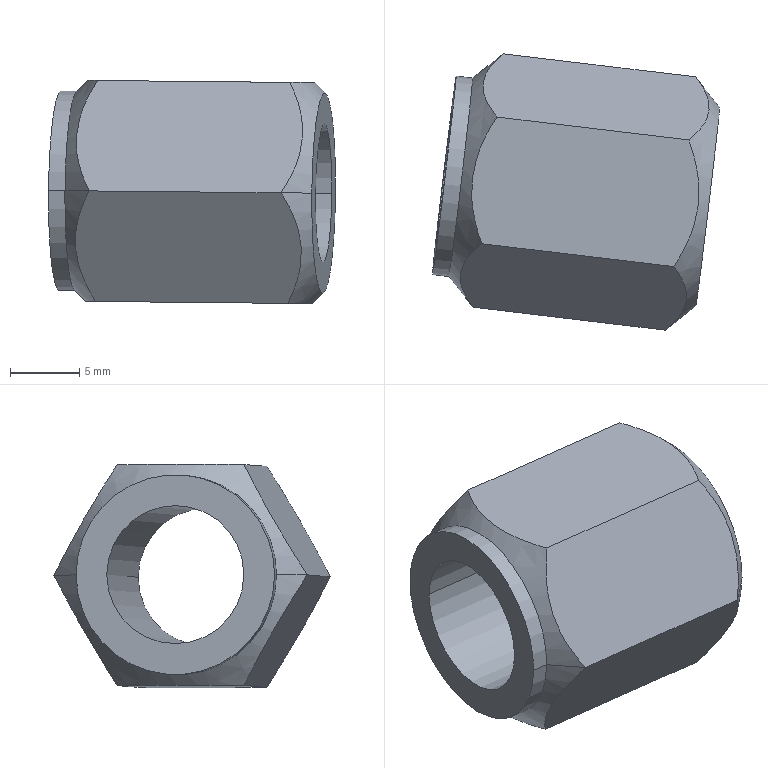Component | SolidWorks | Part13-1 | 1 solid | 16 faces | box 20.78 x 20 x 16.16 mm | volume 2605 mm3 | plane 8 | cone 4 | cylinder 4 | commonest cylinder face diameters 14.475 x2 10 x2 | material 45
build123d program:
from build123d import *

# Parameters (mm, degrees)
SKETCH2_R           = 5
BOSS_EXTRUDE1_DEPTH = 18
SKETCH4_R           = 7.238
SKETCH4_R_2         = 5
BOSS_EXTRUDE2_DEPTH = 1.2


with BuildPart() as part:
    # Sketch2 → Boss-Extrude1 (new body)
    with BuildSketch(Plane.XY):
        Polygon((6.238, 0), (1.619, 8), (-7.619, 8), (-12.238, 0), (-7.619, -8), (1.619, -8), align=None)
        with Locations((-3, 0)):
            Circle(SKETCH2_R, mode=Mode.SUBTRACT)
    extrude(amount=BOSS_EXTRUDE1_DEPTH)

    # Sketch3 → Cut-Revolve1 (revolve, cut)
    with BuildSketch(Plane(origin=(0, 0, 0), x_dir=(1, 0, 0), z_dir=(0, 1, 0)), mode=Mode.PRIVATE) as cut_revolve1_sk:
        Polygon((6.238, -16), (4.238, -18), (6.238, -18), align=None)
    revolve(cut_revolve1_sk.sketch.rotate(Axis((-3, 0, 18), (0, 0, 1)), 180), axis=Axis((-3, 0, 18), (0, 0, 1)), mode=Mode.SUBTRACT)

    # Sketch4 → Boss-Extrude2 (add)
    with BuildSketch(Plane.XY.offset(18)):
        with Locations((-3, 0)):
            Circle(SKETCH4_R)
        with Locations((-3, 0)):
            Circle(SKETCH4_R_2, mode=Mode.SUBTRACT)
    extrude(amount=BOSS_EXTRUDE2_DEPTH)

    # Sketch5 → Cut-Revolve2 (revolve, cut)
    with BuildSketch(Plane(origin=(0, 0, 0), x_dir=(1, 0, 0), z_dir=(0, 1, 0))):
        Polygon((4.238, 0), (6.238, 0), (6.238, -2), align=None)
    revolve(axis=Axis((-3, 0, 0), (0, 0, 1)), mode=Mode.SUBTRACT)


solid = part.part

# Placed as in the assembly
solid = solid.moved(Location((-11.695, 65.586, -1.735), (-85.302, -83.182, -175.339)))
STEP:
#1=COLOUR_RGB('',0.7922,0.8196,0.9333);
#2=FILL_AREA_STYLE_COLOUR('',#1);
#3=FILL_AREA_STYLE('',(#2));
#4=SURFACE_STYLE_FILL_AREA(#3);
#5=SURFACE_SIDE_STYLE('',(#4));
#6=SURFACE_STYLE_USAGE(.BOTH.,#5);
#7=PRESENTATION_STYLE_ASSIGNMENT((#6));
#8=CARTESIAN_POINT('',(-0.4802,2.416,-0.06797));
#9=VERTEX_POINT('',#8);
#10=CARTESIAN_POINT('',(-0.4127,2.982,-0.06863));
#11=VERTEX_POINT('',#10);
#12=CARTESIAN_POINT('',(-0.4465,2.699,-0.0683));
#13=DIRECTION('',(0.9929,-0.1183,-0.009724));
#14=DIRECTION('',(-0.1183,-0.993,0.001159));
#15=AXIS2_PLACEMENT_3D('',#12,#13,#14);
#16=CIRCLE('',#15,0.2849);
#17=EDGE_CURVE('',#9,#11,#16,.T.);
#18=ORIENTED_EDGE('',*,*,#17,.F.);
#19=CARTESIAN_POINT('',(-0.5677,2.348,-0.06712));
#20=VERTEX_POINT('',#19);
#21=CARTESIAN_POINT('',(-0.4802,2.416,-0.06797));
#22=DIRECTION('',(-0.7858,-0.6185,0.007696));
#23=VECTOR('',#22,39.37);
#24=LINE('',#21,#23);
#25=EDGE_CURVE('',#9,#20,#24,.T.);
#26=ORIENTED_EDGE('',*,*,#25,.T.);
#27=CARTESIAN_POINT('',(-0.5492,2.528,-0.3823));
#28=VERTEX_POINT('',#27);
#29=CARTESIAN_POINT('',(-0.5677,2.348,-0.06712));
#30=CARTESIAN_POINT('',(-0.5521,2.36,-0.09188));
#31=CARTESIAN_POINT('',(-0.5387,2.373,-0.1172));
#32=CARTESIAN_POINT('',(-0.5235,2.394,-0.1564));
#33=CARTESIAN_POINT('',(-0.5193,2.401,-0.1697));
#34=CARTESIAN_POINT('',(-0.513,2.416,-0.1969));
#35=CARTESIAN_POINT('',(-0.511,2.424,-0.2108));
#36=CARTESIAN_POINT('',(-0.5084,2.448,-0.2521));
#37=CARTESIAN_POINT('',(-0.5116,2.464,-0.2791));
#38=CARTESIAN_POINT('',(-0.5258,2.496,-0.3323));
#39=CARTESIAN_POINT('',(-0.5365,2.512,-0.3576));
#40=CARTESIAN_POINT('',(-0.5492,2.528,-0.3823));
#41=B_SPLINE_CURVE_WITH_KNOTS('',3,(#29,#30,#31,#32,#33,#34,#35,#36,#37,#38,#39,#40),.UNSPECIFIED.,.F.,.F.,(4,2,2,2,2,4),(0.00000025,0.002386,0.003579,0.004771,0.007157,0.009542),.UNSPECIFIED.);
#42=EDGE_CURVE('',#20,#28,#41,.T.);
#43=ORIENTED_EDGE('',*,*,#42,.T.);
#44=CARTESIAN_POINT('',(-0.5062,2.889,-0.3827));
#45=VERTEX_POINT('',#44);
#46=CARTESIAN_POINT('',(-0.5492,2.528,-0.3823));
#47=CARTESIAN_POINT('',(-0.5406,2.541,-0.3824));
#48=CARTESIAN_POINT('',(-0.5323,2.555,-0.3824));
#49=CARTESIAN_POINT('',(-0.5171,2.583,-0.3826));
#50=CARTESIAN_POINT('',(-0.51,2.597,-0.3827));
#51=CARTESIAN_POINT('',(-0.4979,2.626,-0.3828));
#52=CARTESIAN_POINT('',(-0.4926,2.641,-0.3828));
#53=CARTESIAN_POINT('',(-0.4843,2.671,-0.3829));
#54=CARTESIAN_POINT('',(-0.4812,2.687,-0.3829));
#55=CARTESIAN_POINT('',(-0.4756,2.735,-0.383));
#56=CARTESIAN_POINT('',(-0.4768,2.766,-0.383));
#57=CARTESIAN_POINT('',(-0.4843,2.813,-0.3829));
#58=CARTESIAN_POINT('',(-0.4878,2.829,-0.3829));
#59=CARTESIAN_POINT('',(-0.4961,2.859,-0.3828));
#60=CARTESIAN_POINT('',(-0.5009,2.874,-0.3827));
#61=CARTESIAN_POINT('',(-0.5062,2.889,-0.3827));
#62=B_SPLINE_CURVE_WITH_KNOTS('',3,(#46,#47,#48,#49,#50,#51,#52,#53,#54,#55,#56,#57,#58,#59,#60,#61),.UNSPECIFIED.,.F.,.F.,(4,2,2,2,2,2,2,4),(0.005616,0.006813,0.00801,0.009206,0.0104,0.0128,0.01399,0.01519),.UNSPECIFIED.);
#63=EDGE_CURVE('',#28,#45,#62,.T.);
#64=ORIENTED_EDGE('',*,*,#63,.T.);
#65=CARTESIAN_POINT('',(-0.4816,3.07,-0.06796));
#66=VERTEX_POINT('',#65);
#67=CARTESIAN_POINT('',(-0.5062,2.889,-0.3827));
#68=CARTESIAN_POINT('',(-0.4902,2.902,-0.3582));
#69=CARTESIAN_POINT('',(-0.4762,2.915,-0.3332));
#70=CARTESIAN_POINT('',(-0.4603,2.936,-0.2943));
#71=CARTESIAN_POINT('',(-0.4559,2.943,-0.2811));
#72=CARTESIAN_POINT('',(-0.449,2.958,-0.254));
#73=CARTESIAN_POINT('',(-0.4467,2.966,-0.2401));
#74=CARTESIAN_POINT('',(-0.4434,2.989,-0.1989));
#75=CARTESIAN_POINT('',(-0.446,3.005,-0.1719));
#76=CARTESIAN_POINT('',(-0.4592,3.038,-0.1184));
#77=CARTESIAN_POINT('',(-0.4694,3.054,-0.09283));
#78=CARTESIAN_POINT('',(-0.4816,3.07,-0.06796));
#79=B_SPLINE_CURVE_WITH_KNOTS('',3,(#67,#68,#69,#70,#71,#72,#73,#74,#75,#76,#77,#78),.UNSPECIFIED.,.F.,.F.,(4,2,2,2,2,4),(0.00000025,0.002386,0.003579,0.004771,0.007157,0.009542),.UNSPECIFIED.);
#80=EDGE_CURVE('',#45,#66,#79,.T.);
#81=ORIENTED_EDGE('',*,*,#80,.T.);
#82=CARTESIAN_POINT('',(-0.4127,2.982,-0.06863));
#83=DIRECTION('',(-0.6184,0.7858,0.006057));
#84=VECTOR('',#83,39.37);
#85=LINE('',#82,#84);
#86=EDGE_CURVE('',#11,#66,#85,.T.);
#87=ORIENTED_EDGE('',*,*,#86,.F.);
#88=EDGE_LOOP('',(#18,#26,#43,#64,#81,#87));
#89=FACE_OUTER_BOUND('',#88,.T.);
#90=CARTESIAN_POINT('',(-0.4465,2.699,-0.0683));
#91=DIRECTION('',(-0.9929,0.1183,0.009724));
#92=DIRECTION('',(0.1183,0.993,-0.001159));
#93=AXIS2_PLACEMENT_3D('',#90,#91,#92);
#94=CONICAL_SURFACE('',#93,0.2849,0.7854);
#95=ADVANCED_FACE('',(#89),#94,.T.);
#96=CARTESIAN_POINT('',(-1.163,3.072,-0.06128));
#97=VERTEX_POINT('',#96);
#98=CARTESIAN_POINT('',(-1.231,2.506,-0.06062));
#99=VERTEX_POINT('',#98);
#100=CARTESIAN_POINT('',(-1.197,2.789,-0.06095));
#101=DIRECTION('',(-0.9929,0.1183,0.009724));
#102=DIRECTION('',(0.1183,0.993,-0.001159));
#103=AXIS2_PLACEMENT_3D('',#100,#101,#102);
#104=CIRCLE('',#103,0.2849);
#105=EDGE_CURVE('',#97,#99,#104,.T.);
#106=ORIENTED_EDGE('',*,*,#105,.F.);
#107=CARTESIAN_POINT('',(-1.116,3.066,-0.06174));
#108=VERTEX_POINT('',#107);
#109=CARTESIAN_POINT('',(-1.163,3.072,-0.06128));
#110=DIRECTION('',(0.9929,-0.1183,-0.009724));
#111=VECTOR('',#110,39.37);
#112=LINE('',#109,#111);
#113=EDGE_CURVE('',#97,#108,#112,.T.);
#114=ORIENTED_EDGE('',*,*,#113,.T.);
#115=CARTESIAN_POINT('',(-1.184,2.5,-0.06108));
#116=VERTEX_POINT('',#115);
#117=CARTESIAN_POINT('',(-1.15,2.783,-0.06141));
#118=DIRECTION('',(-0.9929,0.1183,0.009724));
#119=DIRECTION('',(0.1183,0.993,-0.001159));
#120=AXIS2_PLACEMENT_3D('',#117,#118,#119);
#121=CIRCLE('',#120,0.2849);
#122=EDGE_CURVE('',#108,#116,#121,.T.);
#123=ORIENTED_EDGE('',*,*,#122,.T.);
#124=CARTESIAN_POINT('',(-1.231,2.506,-0.06062));
#125=DIRECTION('',(0.9929,-0.1183,-0.009724));
#126=VECTOR('',#125,39.37);
#127=LINE('',#124,#126);
#128=EDGE_CURVE('',#99,#116,#127,.T.);
#129=ORIENTED_EDGE('',*,*,#128,.F.);
#130=EDGE_LOOP('',(#106,#114,#123,#129));
#131=FACE_OUTER_BOUND('',#130,.T.);
#132=CARTESIAN_POINT('',(-1.197,2.789,-0.06095));
#133=DIRECTION('',(0.9929,-0.1183,-0.009724));
#134=DIRECTION('',(-0.1183,-0.993,0.001159));
#135=AXIS2_PLACEMENT_3D('',#132,#133,#134);
#136=CYLINDRICAL_SURFACE('',#135,0.2849);
#137=ADVANCED_FACE('',(#131),#136,.T.);
#138=ORIENTED_EDGE('',*,*,#122,.F.);
#139=CARTESIAN_POINT('',(-1.029,3.135,-0.0626));
#140=VERTEX_POINT('',#139);
#141=CARTESIAN_POINT('',(-1.029,3.135,-0.0626));
#142=DIRECTION('',(0.7858,0.6185,-0.007696));
#143=VECTOR('',#142,39.37);
#144=LINE('',#141,#143);
#145=EDGE_CURVE('',#108,#140,#144,.T.);
#146=ORIENTED_EDGE('',*,*,#145,.T.);
#147=CARTESIAN_POINT('',(-1.053,2.954,-0.3773));
#148=VERTEX_POINT('',#147);
#149=CARTESIAN_POINT('',(-1.029,3.135,-0.0626));
#150=CARTESIAN_POINT('',(-1.045,3.123,-0.08705));
#151=CARTESIAN_POINT('',(-1.059,3.11,-0.1121));
#152=CARTESIAN_POINT('',(-1.075,3.089,-0.151));
#153=CARTESIAN_POINT('',(-1.079,3.082,-0.1642));
#154=CARTESIAN_POINT('',(-1.086,3.067,-0.1913));
#155=CARTESIAN_POINT('',(-1.088,3.059,-0.2052));
#156=CARTESIAN_POINT('',(-1.092,3.035,-0.2464));
#157=CARTESIAN_POINT('',(-1.089,3.019,-0.2734));
#158=CARTESIAN_POINT('',(-1.076,2.986,-0.3269));
#159=CARTESIAN_POINT('',(-1.066,2.97,-0.3525));
#160=CARTESIAN_POINT('',(-1.053,2.954,-0.3773));
#161=B_SPLINE_CURVE_WITH_KNOTS('',3,(#149,#150,#151,#152,#153,#154,#155,#156,#157,#158,#159,#160),.UNSPECIFIED.,.F.,.F.,(4,2,2,2,2,4),(0.00000025,0.002386,0.003579,0.004771,0.007157,0.009542),.UNSPECIFIED.);
#162=EDGE_CURVE('',#140,#148,#161,.T.);
#163=ORIENTED_EDGE('',*,*,#162,.T.);
#164=CARTESIAN_POINT('',(-1.097,2.593,-0.3769));
#165=VERTEX_POINT('',#164);
#166=CARTESIAN_POINT('',(-1.053,2.954,-0.3773));
#167=CARTESIAN_POINT('',(-1.062,2.941,-0.3772));
#168=CARTESIAN_POINT('',(-1.07,2.928,-0.3772));
#169=CARTESIAN_POINT('',(-1.086,2.9,-0.377));
#170=CARTESIAN_POINT('',(-1.093,2.886,-0.3769));
#171=CARTESIAN_POINT('',(-1.111,2.842,-0.3768));
#172=CARTESIAN_POINT('',(-1.12,2.812,-0.3767));
#173=CARTESIAN_POINT('',(-1.125,2.764,-0.3766));
#174=CARTESIAN_POINT('',(-1.126,2.748,-0.3766));
#175=CARTESIAN_POINT('',(-1.125,2.716,-0.3766));
#176=CARTESIAN_POINT('',(-1.123,2.701,-0.3766));
#177=CARTESIAN_POINT('',(-1.118,2.67,-0.3767));
#178=CARTESIAN_POINT('',(-1.115,2.654,-0.3767));
#179=CARTESIAN_POINT('',(-1.107,2.623,-0.3768));
#180=CARTESIAN_POINT('',(-1.102,2.608,-0.3769));
#181=CARTESIAN_POINT('',(-1.097,2.593,-0.3769));
#182=B_SPLINE_CURVE_WITH_KNOTS('',3,(#166,#167,#168,#169,#170,#171,#172,#173,#174,#175,#176,#177,#178,#179,#180,#181),.UNSPECIFIED.,.F.,.F.,(4,2,2,2,2,2,2,4),(0.004981,0.006177,0.007373,0.009765,0.01096,0.01216,0.01335,0.01455),.UNSPECIFIED.);
#183=EDGE_CURVE('',#148,#165,#182,.T.);
#184=ORIENTED_EDGE('',*,*,#183,.T.);
#185=CARTESIAN_POINT('',(-1.115,2.413,-0.06176));
#186=VERTEX_POINT('',#185);
#187=CARTESIAN_POINT('',(-1.097,2.593,-0.3769));
#188=CARTESIAN_POINT('',(-1.112,2.581,-0.3521));
#189=CARTESIAN_POINT('',(-1.126,2.568,-0.3269));
#190=CARTESIAN_POINT('',(-1.141,2.547,-0.2876));
#191=CARTESIAN_POINT('',(-1.145,2.54,-0.2743));
#192=CARTESIAN_POINT('',(-1.151,2.525,-0.2472));
#193=CARTESIAN_POINT('',(-1.153,2.517,-0.2332));
#194=CARTESIAN_POINT('',(-1.156,2.493,-0.1919));
#195=CARTESIAN_POINT('',(-1.153,2.477,-0.1649));
#196=CARTESIAN_POINT('',(-1.138,2.445,-0.1118));
#197=CARTESIAN_POINT('',(-1.128,2.429,-0.08639));
#198=CARTESIAN_POINT('',(-1.115,2.413,-0.06176));
#199=B_SPLINE_CURVE_WITH_KNOTS('',3,(#187,#188,#189,#190,#191,#192,#193,#194,#195,#196,#197,#198),.UNSPECIFIED.,.F.,.F.,(4,2,2,2,2,4),(0.00000025,0.002386,0.003579,0.004771,0.007157,0.009542),.UNSPECIFIED.);
#200=EDGE_CURVE('',#165,#186,#199,.T.);
#201=ORIENTED_EDGE('',*,*,#200,.T.);
#202=CARTESIAN_POINT('',(-1.115,2.413,-0.06176));
#203=DIRECTION('',(0.6184,-0.7858,-0.006057));
#204=VECTOR('',#203,39.37);
#205=LINE('',#202,#204);
#206=EDGE_CURVE('',#116,#186,#205,.T.);
#207=ORIENTED_EDGE('',*,*,#206,.F.);
#208=EDGE_LOOP('',(#138,#146,#163,#184,#201,#207));
#209=FACE_OUTER_BOUND('',#208,.T.);
#210=CARTESIAN_POINT('',(-1.072,2.774,-0.06218));
#211=DIRECTION('',(0.9929,-0.1183,-0.009724));
#212=DIRECTION('',(-0.1183,-0.993,0.001159));
#213=AXIS2_PLACEMENT_3D('',#210,#211,#212);
#214=CONICAL_SURFACE('',#213,0.3637,0.7854);
#215=ADVANCED_FACE('',(#209),#214,.T.);
#216=CARTESIAN_POINT('',(-1.22,2.593,-0.06072));
#217=VERTEX_POINT('',#216);
#218=CARTESIAN_POINT('',(-1.174,2.984,-0.06118));
#219=VERTEX_POINT('',#218);
#220=CARTESIAN_POINT('',(-1.197,2.789,-0.06095));
#221=DIRECTION('',(-0.9929,0.1183,0.009724));
#222=DIRECTION('',(0.1183,0.993,-0.001159));
#223=AXIS2_PLACEMENT_3D('',#220,#221,#222);
#224=CIRCLE('',#223,0.1969);
#225=EDGE_CURVE('',#217,#219,#224,.T.);
#226=ORIENTED_EDGE('',*,*,#225,.T.);
#227=CARTESIAN_POINT('',(-0.4232,2.895,-0.06853));
#228=VERTEX_POINT('',#227);
#229=CARTESIAN_POINT('',(-1.127,2.979,-0.06164));
#230=DIRECTION('',(0.9929,-0.1183,-0.009724));
#231=VECTOR('',#230,39.37);
#232=LINE('',#229,#231);
#233=EDGE_CURVE('',#219,#228,#232,.T.);
#234=ORIENTED_EDGE('',*,*,#233,.T.);
#235=CARTESIAN_POINT('',(-0.4698,2.504,-0.06807));
#236=VERTEX_POINT('',#235);
#237=CARTESIAN_POINT('',(-0.4465,2.699,-0.0683));
#238=DIRECTION('',(-0.9929,0.1183,0.009724));
#239=DIRECTION('',(0.1183,0.993,-0.001159));
#240=AXIS2_PLACEMENT_3D('',#237,#238,#239);
#241=CIRCLE('',#240,0.1969);
#242=EDGE_CURVE('',#236,#228,#241,.T.);
#243=ORIENTED_EDGE('',*,*,#242,.F.);
#244=CARTESIAN_POINT('',(-1.173,2.588,-0.06118));
#245=DIRECTION('',(0.9929,-0.1183,-0.009724));
#246=VECTOR('',#245,39.37);
#247=LINE('',#244,#246);
#248=EDGE_CURVE('',#217,#236,#247,.T.);
#249=ORIENTED_EDGE('',*,*,#248,.F.);
#250=EDGE_LOOP('',(#226,#234,#243,#249));
#251=FACE_OUTER_BOUND('',#250,.T.);
#252=CARTESIAN_POINT('',(-1.15,2.783,-0.06141));
#253=DIRECTION('',(0.9929,-0.1183,-0.009724));
#254=DIRECTION('',(-0.1183,-0.993,0.001159));
#255=AXIS2_PLACEMENT_3D('',#252,#253,#254);
#256=CYLINDRICAL_SURFACE('',#255,0.1969);
#257=ADVANCED_FACE('',(#251),#256,.F.);
#258=CARTESIAN_POINT('',(-0.5,2.889,0.2472));
#259=VERTEX_POINT('',#258);
#260=CARTESIAN_POINT('',(-0.4816,3.07,-0.06796));
#261=CARTESIAN_POINT('',(-0.4689,3.054,-0.04347));
#262=CARTESIAN_POINT('',(-0.4584,3.038,-0.01841));
#263=CARTESIAN_POINT('',(-0.4479,3.014,0.02058));
#264=CARTESIAN_POINT('',(-0.4452,3.006,0.03382));
#265=CARTESIAN_POINT('',(-0.4421,2.99,0.06087));
#266=CARTESIAN_POINT('',(-0.4416,2.982,0.07481));
#267=CARTESIAN_POINT('',(-0.444,2.958,0.1161));
#268=CARTESIAN_POINT('',(-0.4503,2.943,0.1432));
#269=CARTESIAN_POINT('',(-0.4707,2.915,0.1967));
#270=CARTESIAN_POINT('',(-0.4844,2.902,0.2223));
#271=CARTESIAN_POINT('',(-0.5,2.889,0.2472));
#272=B_SPLINE_CURVE_WITH_KNOTS('',3,(#260,#261,#262,#263,#264,#265,#266,#267,#268,#269,#270,#271),.UNSPECIFIED.,.F.,.F.,(4,2,2,2,2,4),(0.00000025,0.002386,0.003579,0.004771,0.007157,0.009542),.UNSPECIFIED.);
#273=EDGE_CURVE('',#66,#259,#272,.T.);
#274=ORIENTED_EDGE('',*,*,#273,.F.);
#275=CARTESIAN_POINT('',(-1.107,3.144,-0.06183));
#276=DIRECTION('',(0.9929,-0.1183,-0.009724));
#277=VECTOR('',#276,39.37);
#278=LINE('',#275,#277);
#279=EDGE_CURVE('',#140,#66,#278,.T.);
#280=ORIENTED_EDGE('',*,*,#279,.F.);
#281=CARTESIAN_POINT('',(-1.047,2.954,0.2526));
#282=VERTEX_POINT('',#281);
#283=CARTESIAN_POINT('',(-1.047,2.954,0.2526));
#284=CARTESIAN_POINT('',(-1.06,2.97,0.2281));
#285=CARTESIAN_POINT('',(-1.071,2.986,0.203));
#286=CARTESIAN_POINT('',(-1.081,3.01,0.164));
#287=CARTESIAN_POINT('',(-1.084,3.018,0.1508));
#288=CARTESIAN_POINT('',(-1.087,3.034,0.1237));
#289=CARTESIAN_POINT('',(-1.087,3.042,0.1098));
#290=CARTESIAN_POINT('',(-1.085,3.066,0.06852));
#291=CARTESIAN_POINT('',(-1.079,3.081,0.04143));
#292=CARTESIAN_POINT('',(-1.058,3.109,-0.01207));
#293=CARTESIAN_POINT('',(-1.045,3.123,-0.03769));
#294=CARTESIAN_POINT('',(-1.029,3.135,-0.0626));
#295=B_SPLINE_CURVE_WITH_KNOTS('',3,(#283,#284,#285,#286,#287,#288,#289,#290,#291,#292,#293,#294),.UNSPECIFIED.,.F.,.F.,(4,2,2,2,2,4),(0.00000025,0.002386,0.003579,0.004771,0.007157,0.009542),.UNSPECIFIED.);
#296=EDGE_CURVE('',#282,#140,#295,.T.);
#297=ORIENTED_EDGE('',*,*,#296,.F.);
#298=CARTESIAN_POINT('',(-1.126,2.964,0.2533));
#299=DIRECTION('',(0.9929,-0.1183,-0.009724));
#300=VECTOR('',#299,39.37);
#301=LINE('',#298,#300);
#302=EDGE_CURVE('',#282,#259,#301,.T.);
#303=ORIENTED_EDGE('',*,*,#302,.T.);
#304=EDGE_LOOP('',(#274,#280,#297,#303));
#305=FACE_OUTER_BOUND('',#304,.T.);
#306=CARTESIAN_POINT('',(-1.126,2.964,0.2533));
#307=DIRECTION('',(-0.1074,-0.8599,-0.499));
#308=DIRECTION('',(-0.05068,-0.4965,0.8666));
#309=AXIS2_PLACEMENT_3D('',#306,#307,#308);
#310=PLANE('',#309);
#311=ADVANCED_FACE('',(#305),#310,.F.);
#312=ORIENTED_EDGE('',*,*,#80,.F.);
#313=CARTESIAN_POINT('',(-1.132,2.964,-0.3766));
#314=DIRECTION('',(0.9929,-0.1183,-0.009724));
#315=VECTOR('',#314,39.37);
#316=LINE('',#313,#315);
#317=EDGE_CURVE('',#148,#45,#316,.T.);
#318=ORIENTED_EDGE('',*,*,#317,.F.);
#319=ORIENTED_EDGE('',*,*,#162,.F.);
#320=ORIENTED_EDGE('',*,*,#279,.T.);
#321=EDGE_LOOP('',(#312,#318,#319,#320));
#322=FACE_OUTER_BOUND('',#321,.T.);
#323=CARTESIAN_POINT('',(-1.107,3.144,-0.06183));
#324=DIRECTION('',(-0.09757,-0.8599,0.501));
#325=DIRECTION('',(0.06764,0.4965,0.8654));
#326=AXIS2_PLACEMENT_3D('',#323,#324,#325);
#327=PLANE('',#326);
#328=ADVANCED_FACE('',(#322),#327,.F.);
#329=ORIENTED_EDGE('',*,*,#63,.F.);
#330=CARTESIAN_POINT('',(-1.175,2.603,-0.3761));
#331=DIRECTION('',(0.9929,-0.1183,-0.009724));
#332=VECTOR('',#331,39.37);
#333=LINE('',#330,#332);
#334=EDGE_CURVE('',#165,#28,#333,.T.);
#335=ORIENTED_EDGE('',*,*,#334,.F.);
#336=ORIENTED_EDGE('',*,*,#183,.F.);
#337=ORIENTED_EDGE('',*,*,#317,.T.);
#338=EDGE_LOOP('',(#329,#335,#336,#337));
#339=FACE_OUTER_BOUND('',#338,.T.);
#340=CARTESIAN_POINT('',(-1.132,2.964,-0.3766));
#341=DIRECTION('',(0.009793,0.,1.));
#342=DIRECTION('',(0.9929,-0.1183,-0.009724));
#343=AXIS2_PLACEMENT_3D('',#340,#341,#342);
#344=PLANE('',#343);
#345=ADVANCED_FACE('',(#339),#344,.F.);
#346=ORIENTED_EDGE('',*,*,#42,.F.);
#347=CARTESIAN_POINT('',(-1.193,2.422,-0.06099));
#348=DIRECTION('',(0.9929,-0.1183,-0.009724));
#349=VECTOR('',#348,39.37);
#350=LINE('',#347,#349);
#351=EDGE_CURVE('',#186,#20,#350,.T.);
#352=ORIENTED_EDGE('',*,*,#351,.F.);
#353=ORIENTED_EDGE('',*,*,#200,.F.);
#354=ORIENTED_EDGE('',*,*,#334,.T.);
#355=EDGE_LOOP('',(#346,#352,#353,#354));
#356=FACE_OUTER_BOUND('',#355,.T.);
#357=CARTESIAN_POINT('',(-1.175,2.603,-0.3761));
#358=DIRECTION('',(0.1074,0.8599,0.499));
#359=DIRECTION('',(0.05068,0.4965,-0.8666));
#360=AXIS2_PLACEMENT_3D('',#357,#358,#359);
#361=PLANE('',#360);
#362=ADVANCED_FACE('',(#356),#361,.F.);
#363=CARTESIAN_POINT('',(-0.5431,2.528,0.2476));
#364=VERTEX_POINT('',#363);
#365=CARTESIAN_POINT('',(-0.5431,2.528,0.2476));
#366=CARTESIAN_POINT('',(-0.5309,2.512,0.2229));
#367=CARTESIAN_POINT('',(-0.5209,2.497,0.1976));
#368=CARTESIAN_POINT('',(-0.5111,2.473,0.1584));
#369=CARTESIAN_POINT('',(-0.5087,2.465,0.1451));
#370=CARTESIAN_POINT('',(-0.5061,2.448,0.118));
#371=CARTESIAN_POINT('',(-0.5059,2.44,0.1041));
#372=CARTESIAN_POINT('',(-0.509,2.417,0.06288));
#373=CARTESIAN_POINT('',(-0.5159,2.402,0.03592));
#374=CARTESIAN_POINT('',(-0.5374,2.373,-0.01717));
#375=CARTESIAN_POINT('',(-0.5516,2.36,-0.04252));
#376=CARTESIAN_POINT('',(-0.5677,2.348,-0.06712));
#377=B_SPLINE_CURVE_WITH_KNOTS('',3,(#365,#366,#367,#368,#369,#370,#371,#372,#373,#374,#375,#376),.UNSPECIFIED.,.F.,.F.,(4,2,2,2,2,4),(0.00000025,0.002386,0.003579,0.004771,0.007157,0.009542),.UNSPECIFIED.);
#378=EDGE_CURVE('',#364,#20,#377,.T.);
#379=ORIENTED_EDGE('',*,*,#378,.F.);
#380=CARTESIAN_POINT('',(-1.09,2.593,0.253));
#381=VERTEX_POINT('',#380);
#382=CARTESIAN_POINT('',(-1.169,2.603,0.2537));
#383=DIRECTION('',(0.9929,-0.1183,-0.009724));
#384=VECTOR('',#383,39.37);
#385=LINE('',#382,#384);
#386=EDGE_CURVE('',#381,#364,#385,.T.);
#387=ORIENTED_EDGE('',*,*,#386,.F.);
#388=CARTESIAN_POINT('',(-1.115,2.413,-0.06176));
#389=CARTESIAN_POINT('',(-1.127,2.429,-0.03703));
#390=CARTESIAN_POINT('',(-1.137,2.444,-0.01176));
#391=CARTESIAN_POINT('',(-1.147,2.468,0.02743));
#392=CARTESIAN_POINT('',(-1.149,2.476,0.04071));
#393=CARTESIAN_POINT('',(-1.152,2.492,0.06782));
#394=CARTESIAN_POINT('',(-1.152,2.501,0.08177));
#395=CARTESIAN_POINT('',(-1.149,2.524,0.123));
#396=CARTESIAN_POINT('',(-1.142,2.539,0.1499));
#397=CARTESIAN_POINT('',(-1.121,2.568,0.203));
#398=CARTESIAN_POINT('',(-1.106,2.581,0.2284));
#399=CARTESIAN_POINT('',(-1.09,2.593,0.253));
#400=B_SPLINE_CURVE_WITH_KNOTS('',3,(#388,#389,#390,#391,#392,#393,#394,#395,#396,#397,#398,#399),.UNSPECIFIED.,.F.,.F.,(4,2,2,2,2,4),(0.00000025,0.002386,0.003579,0.004771,0.007157,0.009542),.UNSPECIFIED.);
#401=EDGE_CURVE('',#186,#381,#400,.T.);
#402=ORIENTED_EDGE('',*,*,#401,.F.);
#403=ORIENTED_EDGE('',*,*,#351,.T.);
#404=EDGE_LOOP('',(#379,#387,#402,#403));
#405=FACE_OUTER_BOUND('',#404,.T.);
#406=CARTESIAN_POINT('',(-1.193,2.422,-0.06099));
#407=DIRECTION('',(0.09757,0.8599,-0.501));
#408=DIRECTION('',(-0.06764,-0.4965,-0.8654));
#409=AXIS2_PLACEMENT_3D('',#406,#407,#408);
#410=PLANE('',#409);
#411=ADVANCED_FACE('',(#405),#410,.F.);
#412=CARTESIAN_POINT('',(-0.5,2.889,0.2472));
#413=CARTESIAN_POINT('',(-0.4947,2.874,0.2471));
#414=CARTESIAN_POINT('',(-0.4899,2.859,0.2471));
#415=CARTESIAN_POINT('',(-0.4816,2.829,0.247));
#416=CARTESIAN_POINT('',(-0.4781,2.813,0.247));
#417=CARTESIAN_POINT('',(-0.4706,2.766,0.2469));
#418=CARTESIAN_POINT('',(-0.4694,2.735,0.2469));
#419=CARTESIAN_POINT('',(-0.4751,2.687,0.247));
#420=CARTESIAN_POINT('',(-0.4782,2.671,0.247));
#421=CARTESIAN_POINT('',(-0.4865,2.641,0.2471));
#422=CARTESIAN_POINT('',(-0.4917,2.626,0.2471));
#423=CARTESIAN_POINT('',(-0.5039,2.597,0.2472));
#424=CARTESIAN_POINT('',(-0.5109,2.583,0.2473));
#425=CARTESIAN_POINT('',(-0.5262,2.555,0.2475));
#426=CARTESIAN_POINT('',(-0.5344,2.541,0.2475));
#427=CARTESIAN_POINT('',(-0.5431,2.528,0.2476));
#428=B_SPLINE_CURVE_WITH_KNOTS('',3,(#412,#413,#414,#415,#416,#417,#418,#419,#420,#421,#422,#423,#424,#425,#426,#427),.UNSPECIFIED.,.F.,.F.,(4,2,2,2,2,2,2,4),(0.004981,0.006177,0.007373,0.009765,0.01096,0.01216,0.01335,0.01455),.UNSPECIFIED.);
#429=EDGE_CURVE('',#259,#364,#428,.T.);
#430=ORIENTED_EDGE('',*,*,#429,.F.);
#431=ORIENTED_EDGE('',*,*,#302,.F.);
#432=CARTESIAN_POINT('',(-1.09,2.593,0.253));
#433=CARTESIAN_POINT('',(-1.096,2.608,0.253));
#434=CARTESIAN_POINT('',(-1.101,2.623,0.2531));
#435=CARTESIAN_POINT('',(-1.109,2.654,0.2532));
#436=CARTESIAN_POINT('',(-1.112,2.67,0.2532));
#437=CARTESIAN_POINT('',(-1.117,2.701,0.2532));
#438=CARTESIAN_POINT('',(-1.119,2.716,0.2533));
#439=CARTESIAN_POINT('',(-1.12,2.748,0.2533));
#440=CARTESIAN_POINT('',(-1.119,2.764,0.2533));
#441=CARTESIAN_POINT('',(-1.113,2.812,0.2532));
#442=CARTESIAN_POINT('',(-1.105,2.842,0.2531));
#443=CARTESIAN_POINT('',(-1.086,2.886,0.2529));
#444=CARTESIAN_POINT('',(-1.079,2.9,0.2529));
#445=CARTESIAN_POINT('',(-1.064,2.928,0.2527));
#446=CARTESIAN_POINT('',(-1.056,2.941,0.2526));
#447=CARTESIAN_POINT('',(-1.047,2.954,0.2526));
#448=B_SPLINE_CURVE_WITH_KNOTS('',3,(#432,#433,#434,#435,#436,#437,#438,#439,#440,#441,#442,#443,#444,#445,#446,#447),.UNSPECIFIED.,.F.,.F.,(4,2,2,2,2,2,2,4),(0.005616,0.006813,0.00801,0.009206,0.0104,0.0128,0.01399,0.01519),.UNSPECIFIED.);
#449=EDGE_CURVE('',#381,#282,#448,.T.);
#450=ORIENTED_EDGE('',*,*,#449,.F.);
#451=ORIENTED_EDGE('',*,*,#386,.T.);
#452=EDGE_LOOP('',(#430,#431,#450,#451));
#453=FACE_OUTER_BOUND('',#452,.T.);
#454=CARTESIAN_POINT('',(-1.169,2.603,0.2537));
#455=DIRECTION('',(-0.009793,-0.,-1.));
#456=DIRECTION('',(-0.9929,0.1183,0.009724));
#457=AXIS2_PLACEMENT_3D('',#454,#455,#456);
#458=PLANE('',#457);
#459=ADVANCED_FACE('',(#453),#458,.F.);
#460=ORIENTED_EDGE('',*,*,#242,.T.);
#461=CARTESIAN_POINT('',(-0.4465,2.699,-0.0683));
#462=DIRECTION('',(-0.9929,0.1183,0.009724));
#463=DIRECTION('',(0.1183,0.993,-0.001159));
#464=AXIS2_PLACEMENT_3D('',#461,#462,#463);
#465=CIRCLE('',#464,0.1969);
#466=EDGE_CURVE('',#228,#236,#465,.T.);
#467=ORIENTED_EDGE('',*,*,#466,.T.);
#468=EDGE_LOOP('',(#460,#467));
#469=FACE_BOUND('',#468,.T.);
#470=CARTESIAN_POINT('',(-0.4465,2.699,-0.0683));
#471=DIRECTION('',(0.9929,-0.1183,-0.009724));
#472=DIRECTION('',(-0.1183,-0.993,0.001159));
#473=AXIS2_PLACEMENT_3D('',#470,#471,#472);
#474=CIRCLE('',#473,0.2849);
#475=EDGE_CURVE('',#11,#9,#474,.T.);
#476=ORIENTED_EDGE('',*,*,#475,.T.);
#477=ORIENTED_EDGE('',*,*,#17,.T.);
#478=EDGE_LOOP('',(#476,#477));
#479=FACE_OUTER_BOUND('',#478,.T.);
#480=CARTESIAN_POINT('',(-0.4325,2.817,-0.06844));
#481=DIRECTION('',(-0.9929,0.1183,0.009724));
#482=DIRECTION('',(0.1183,0.993,-0.001159));
#483=AXIS2_PLACEMENT_3D('',#480,#481,#482);
#484=PLANE('',#483);
#485=ADVANCED_FACE('',(#469,#479),#484,.F.);
#486=ORIENTED_EDGE('',*,*,#233,.F.);
#487=CARTESIAN_POINT('',(-1.197,2.789,-0.06095));
#488=DIRECTION('',(-0.9929,0.1183,0.009724));
#489=DIRECTION('',(0.1183,0.993,-0.001159));
#490=AXIS2_PLACEMENT_3D('',#487,#488,#489);
#491=CIRCLE('',#490,0.1969);
#492=EDGE_CURVE('',#219,#217,#491,.T.);
#493=ORIENTED_EDGE('',*,*,#492,.T.);
#494=ORIENTED_EDGE('',*,*,#248,.T.);
#495=ORIENTED_EDGE('',*,*,#466,.F.);
#496=EDGE_LOOP('',(#486,#493,#494,#495));
#497=FACE_OUTER_BOUND('',#496,.T.);
#498=CARTESIAN_POINT('',(-1.15,2.783,-0.06141));
#499=DIRECTION('',(0.9929,-0.1183,-0.009724));
#500=DIRECTION('',(-0.1183,-0.993,0.001159));
#501=AXIS2_PLACEMENT_3D('',#498,#499,#500);
#502=CYLINDRICAL_SURFACE('',#501,0.1969);
#503=ADVANCED_FACE('',(#497),#502,.F.);
#504=ORIENTED_EDGE('',*,*,#145,.F.);
#505=CARTESIAN_POINT('',(-1.15,2.783,-0.06141));
#506=DIRECTION('',(-0.9929,0.1183,0.009724));
#507=DIRECTION('',(0.1183,0.993,-0.001159));
#508=AXIS2_PLACEMENT_3D('',#505,#506,#507);
#509=CIRCLE('',#508,0.2849);
#510=EDGE_CURVE('',#116,#108,#509,.T.);
#511=ORIENTED_EDGE('',*,*,#510,.F.);
#512=ORIENTED_EDGE('',*,*,#206,.T.);
#513=ORIENTED_EDGE('',*,*,#401,.T.);
#514=ORIENTED_EDGE('',*,*,#449,.T.);
#515=ORIENTED_EDGE('',*,*,#296,.T.);
#516=EDGE_LOOP('',(#504,#511,#512,#513,#514,#515));
#517=FACE_OUTER_BOUND('',#516,.T.);
#518=CARTESIAN_POINT('',(-1.072,2.774,-0.06218));
#519=DIRECTION('',(0.9929,-0.1183,-0.009724));
#520=DIRECTION('',(-0.1183,-0.993,0.001159));
#521=AXIS2_PLACEMENT_3D('',#518,#519,#520);
#522=CONICAL_SURFACE('',#521,0.3637,0.7854);
#523=ADVANCED_FACE('',(#517),#522,.T.);
#524=CARTESIAN_POINT('',(-1.197,2.789,-0.06095));
#525=DIRECTION('',(-0.9929,0.1183,0.009724));
#526=DIRECTION('',(0.1183,0.993,-0.001159));
#527=AXIS2_PLACEMENT_3D('',#524,#525,#526);
#528=CIRCLE('',#527,0.2849);
#529=EDGE_CURVE('',#99,#97,#528,.T.);
#530=ORIENTED_EDGE('',*,*,#529,.T.);
#531=ORIENTED_EDGE('',*,*,#105,.T.);
#532=EDGE_LOOP('',(#530,#531));
#533=FACE_OUTER_BOUND('',#532,.T.);
#534=ORIENTED_EDGE('',*,*,#225,.F.);
#535=ORIENTED_EDGE('',*,*,#492,.F.);
#536=EDGE_LOOP('',(#534,#535));
#537=FACE_BOUND('',#536,.T.);
#538=CARTESIAN_POINT('',(-1.197,2.789,-0.06095));
#539=DIRECTION('',(-0.9929,0.1183,0.009724));
#540=DIRECTION('',(0.1183,0.993,-0.001159));
#541=AXIS2_PLACEMENT_3D('',#538,#539,#540);
#542=PLANE('',#541);
#543=ADVANCED_FACE('',(#533,#537),#542,.T.);
#544=ORIENTED_EDGE('',*,*,#113,.F.);
#545=ORIENTED_EDGE('',*,*,#529,.F.);
#546=ORIENTED_EDGE('',*,*,#128,.T.);
#547=ORIENTED_EDGE('',*,*,#510,.T.);
#548=EDGE_LOOP('',(#544,#545,#546,#547));
#549=FACE_OUTER_BOUND('',#548,.T.);
#550=CARTESIAN_POINT('',(-1.197,2.789,-0.06095));
#551=DIRECTION('',(0.9929,-0.1183,-0.009724));
#552=DIRECTION('',(-0.1183,-0.993,0.001159));
#553=AXIS2_PLACEMENT_3D('',#550,#551,#552);
#554=CYLINDRICAL_SURFACE('',#553,0.2849);
#555=ADVANCED_FACE('',(#549),#554,.T.);
#556=ORIENTED_EDGE('',*,*,#25,.F.);
#557=ORIENTED_EDGE('',*,*,#475,.F.);
#558=ORIENTED_EDGE('',*,*,#86,.T.);
#559=ORIENTED_EDGE('',*,*,#273,.T.);
#560=ORIENTED_EDGE('',*,*,#429,.T.);
#561=ORIENTED_EDGE('',*,*,#378,.T.);
#562=EDGE_LOOP('',(#556,#557,#558,#559,#560,#561));
#563=FACE_OUTER_BOUND('',#562,.T.);
#564=CARTESIAN_POINT('',(-0.4465,2.699,-0.0683));
#565=DIRECTION('',(-0.9929,0.1183,0.009724));
#566=DIRECTION('',(0.1183,0.993,-0.001159));
#567=AXIS2_PLACEMENT_3D('',#564,#565,#566);
#568=CONICAL_SURFACE('',#567,0.2849,0.7854);
#569=ADVANCED_FACE('',(#563),#568,.T.);
#570=CLOSED_SHELL('',(#95,#137,#215,#257,#311,#328,#345,#362,#411,#459,#485,#503,#523,#543,#555,#569));
#571=MANIFOLD_SOLID_BREP('',#570);
#572=STYLED_ITEM('',(#7),#571);
#573=(LENGTH_UNIT()NAMED_UNIT(*)SI_UNIT($,.METRE.));
#574=LENGTH_MEASURE_WITH_UNIT(LENGTH_MEASURE(0.0254),#573);
#575=DIMENSIONAL_EXPONENTS(1.,0.,0.,0.,0.,0.,0.);
#576=(CONVERSION_BASED_UNIT('',#574)LENGTH_UNIT()NAMED_UNIT(#575));
#577=UNCERTAINTY_MEASURE_WITH_UNIT(LENGTH_MEASURE(0.00001),#576,'','');
#578=(NAMED_UNIT(*)PLANE_ANGLE_UNIT()SI_UNIT($,.RADIAN.));
#579=(NAMED_UNIT(*)SI_UNIT($,.STERADIAN.)SOLID_ANGLE_UNIT());
#580=(GEOMETRIC_REPRESENTATION_CONTEXT(3)GLOBAL_UNCERTAINTY_ASSIGNED_CONTEXT((#577))GLOBAL_UNIT_ASSIGNED_CONTEXT((#576,#578,#579))REPRESENTATION_CONTEXT('',''));
#581=MECHANICAL_DESIGN_GEOMETRIC_PRESENTATION_REPRESENTATION('',(#572),#580);
#582=PRESENTATION_LAYER_ASSIGNMENT('','',(#572));
#583=CARTESIAN_POINT('',(0.,0.,0.));
#584=DIRECTION('',(0.,0.,1.));
#585=DIRECTION('',(1.,0.,0.));
#586=AXIS2_PLACEMENT_3D('',#583,#584,#585);
#587=(LENGTH_UNIT()NAMED_UNIT(*)SI_UNIT($,.METRE.));
#588=LENGTH_MEASURE_WITH_UNIT(LENGTH_MEASURE(0.0254),#587);
#589=DIMENSIONAL_EXPONENTS(1.,0.,0.,0.,0.,0.,0.);
#590=(CONVERSION_BASED_UNIT('',#588)LENGTH_UNIT()NAMED_UNIT(#589));
#591=UNCERTAINTY_MEASURE_WITH_UNIT(LENGTH_MEASURE(0.00001),#590,'','');
#592=(NAMED_UNIT(*)PLANE_ANGLE_UNIT()SI_UNIT($,.RADIAN.));
#593=(NAMED_UNIT(*)SI_UNIT($,.STERADIAN.)SOLID_ANGLE_UNIT());
#594=(GEOMETRIC_REPRESENTATION_CONTEXT(3)GLOBAL_UNCERTAINTY_ASSIGNED_CONTEXT((#591))GLOBAL_UNIT_ASSIGNED_CONTEXT((#590,#592,#593))REPRESENTATION_CONTEXT('',''));
#595=ADVANCED_BREP_SHAPE_REPRESENTATION('',(#571,#586),#594);